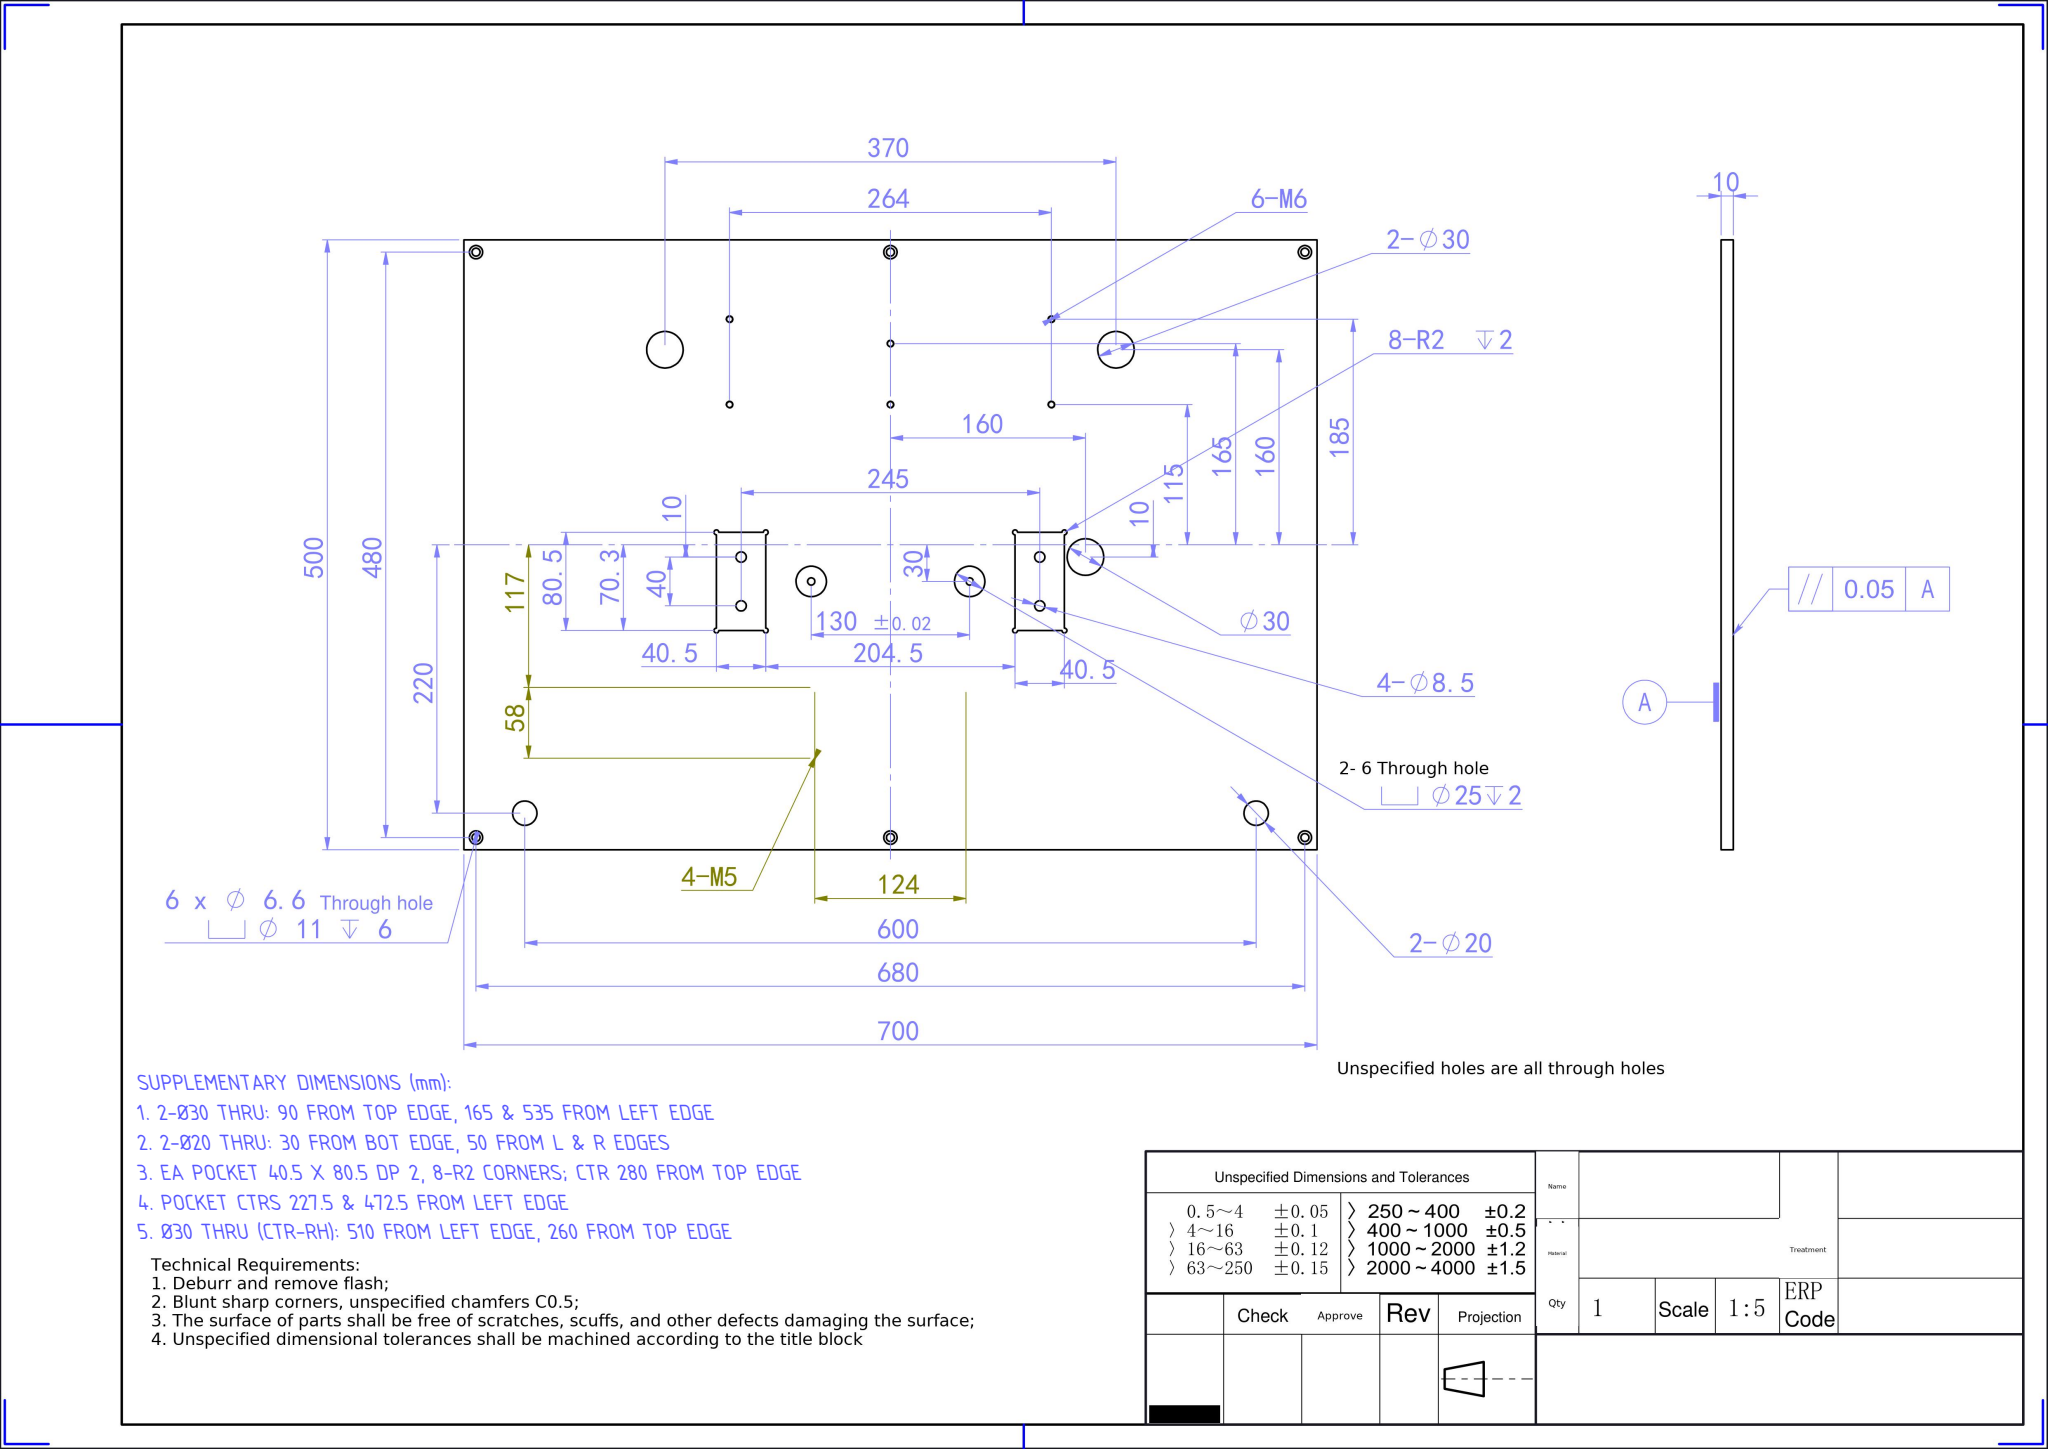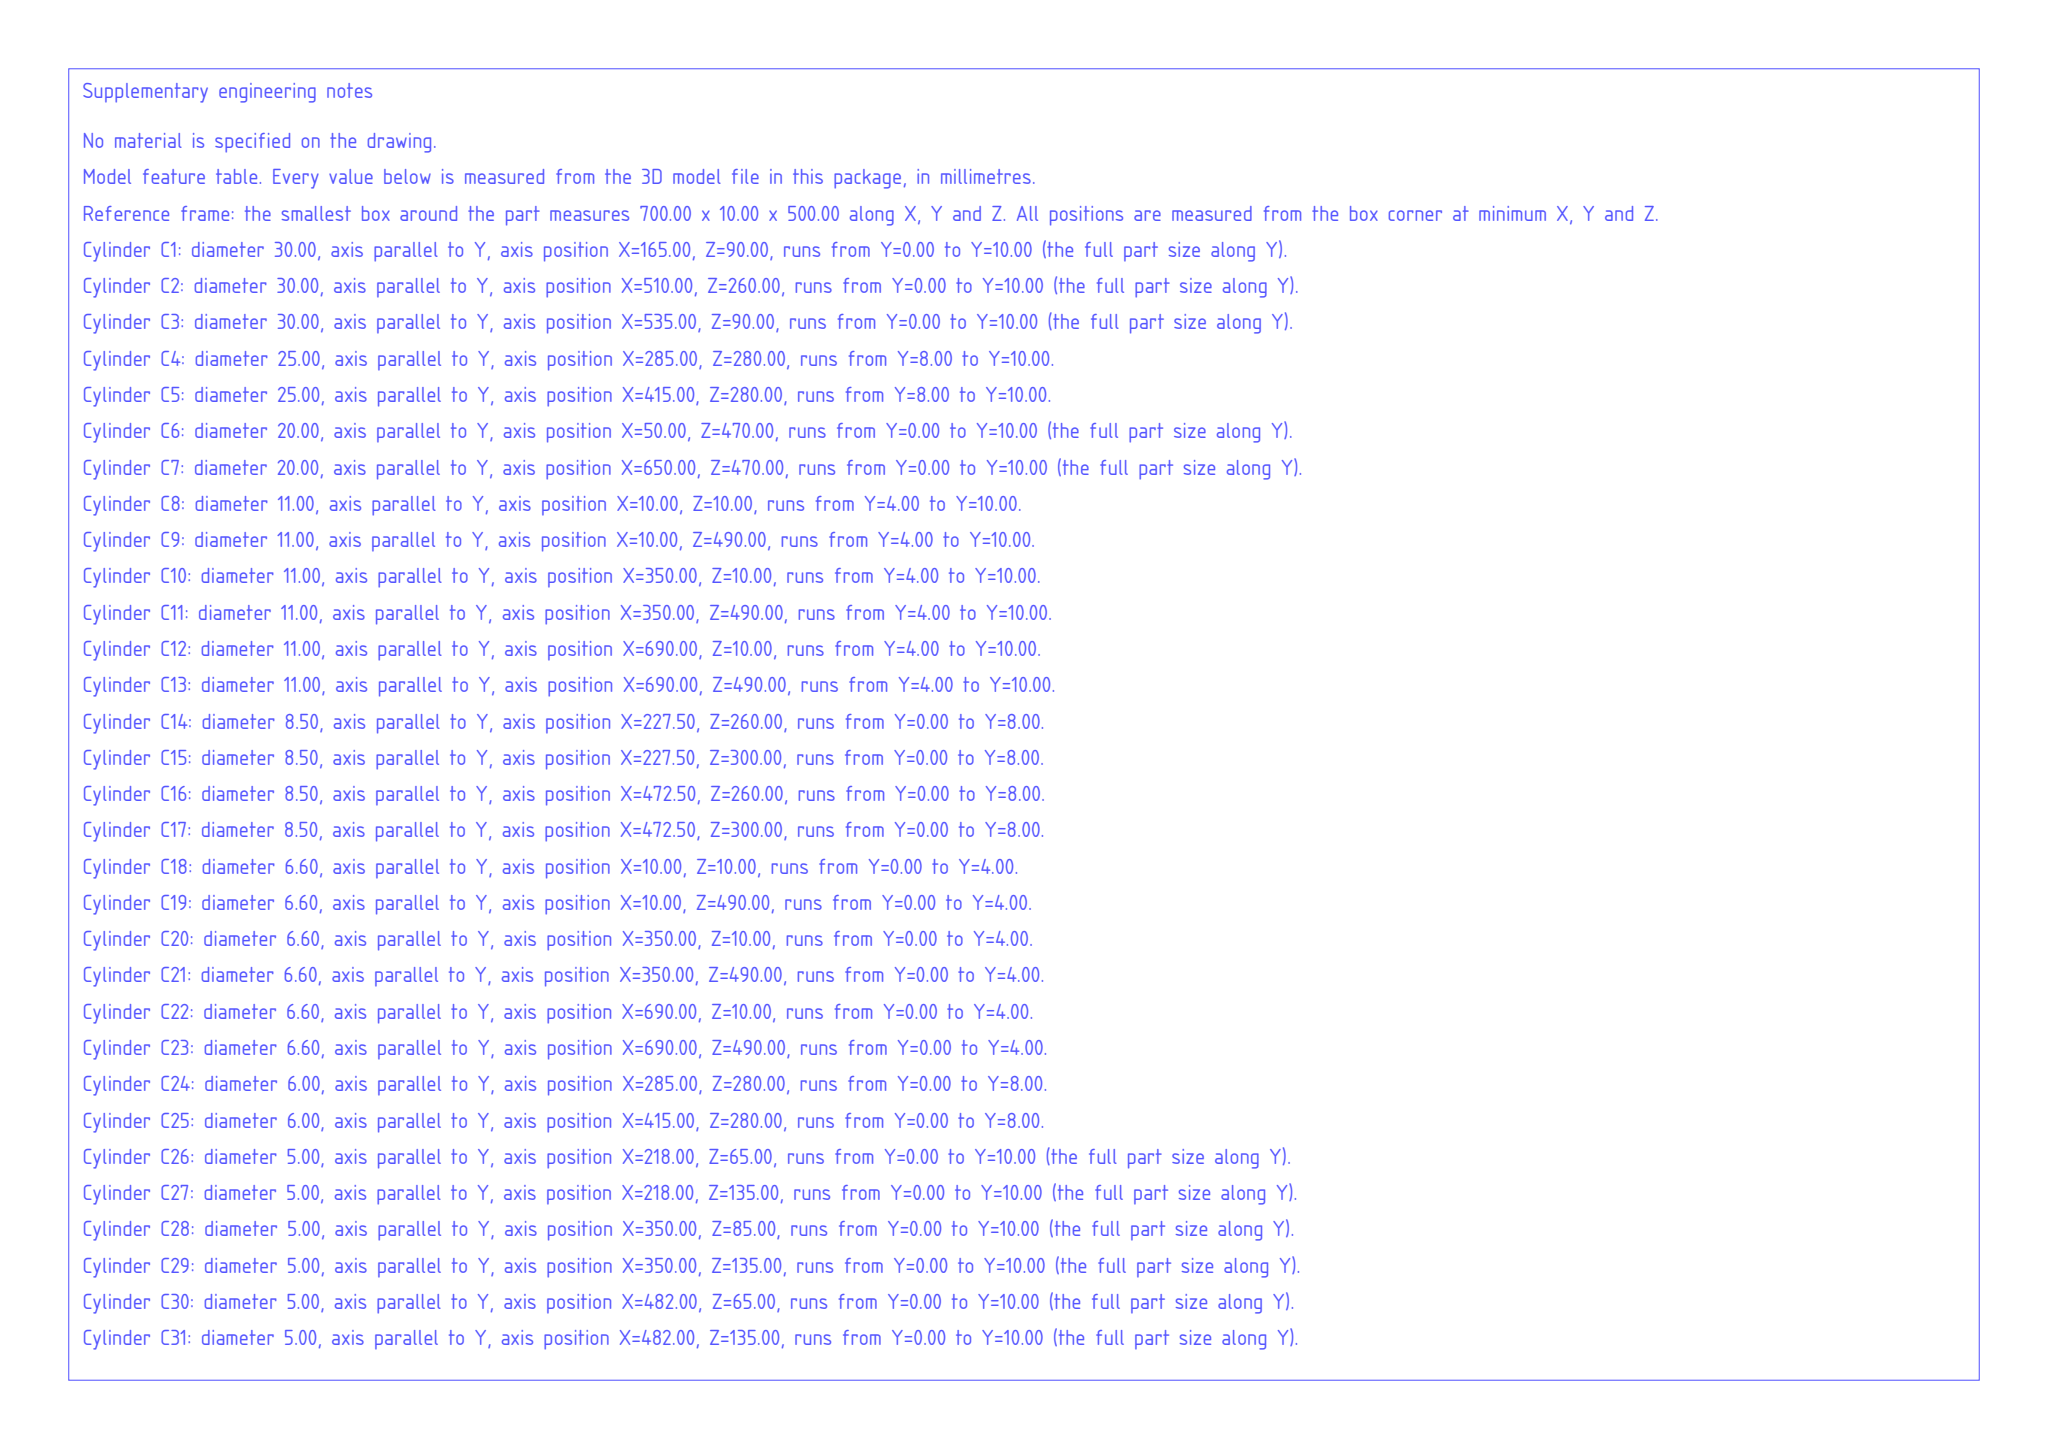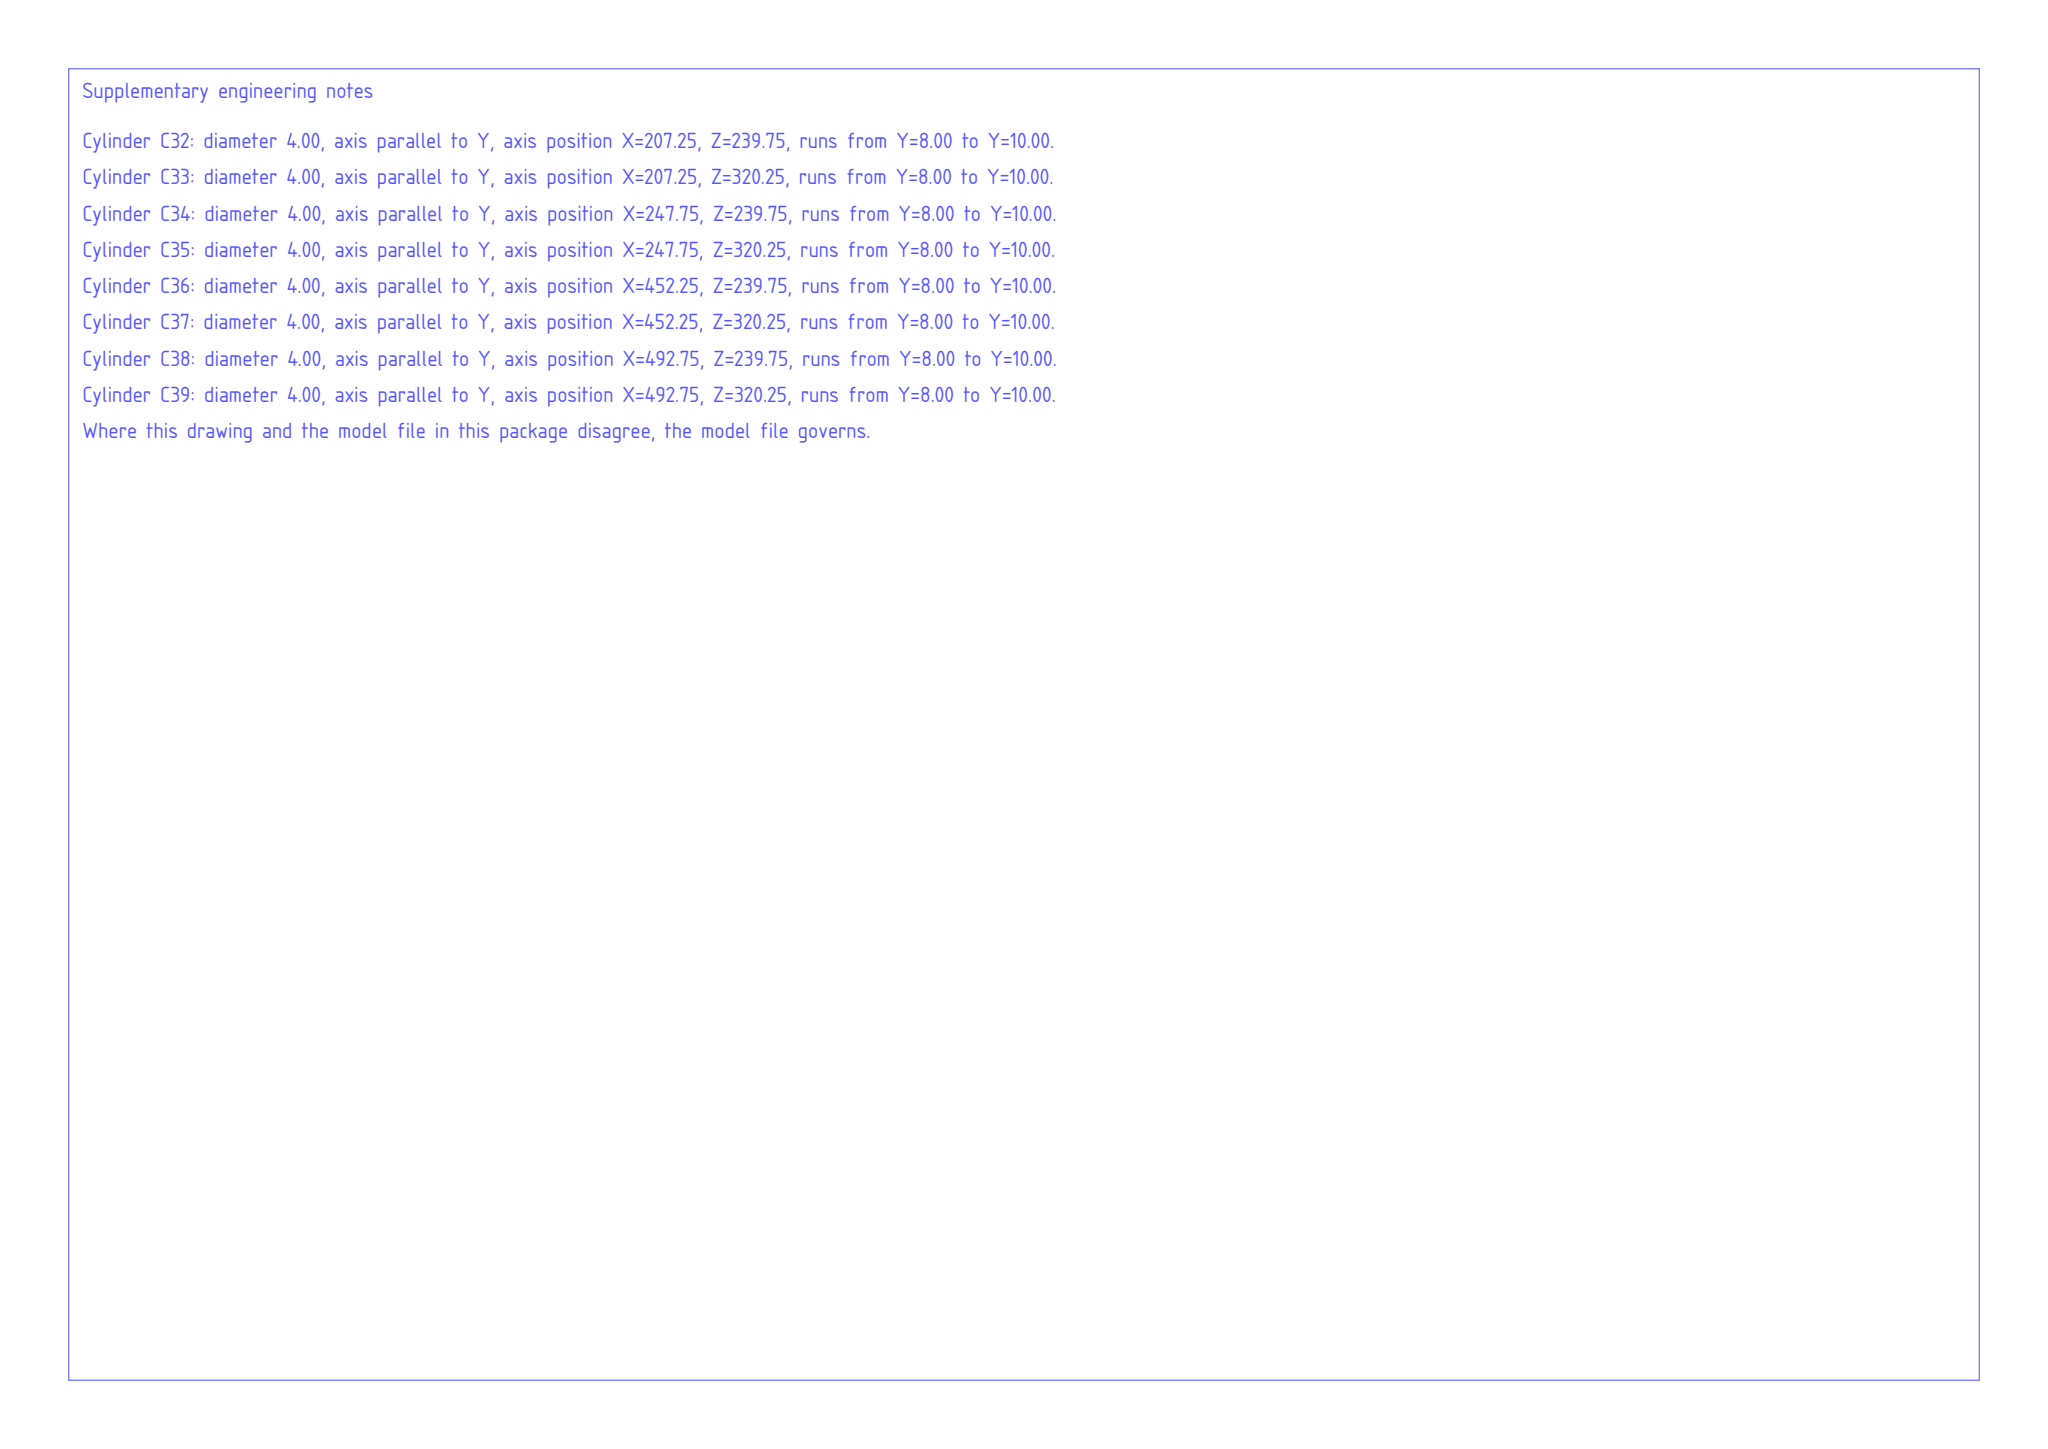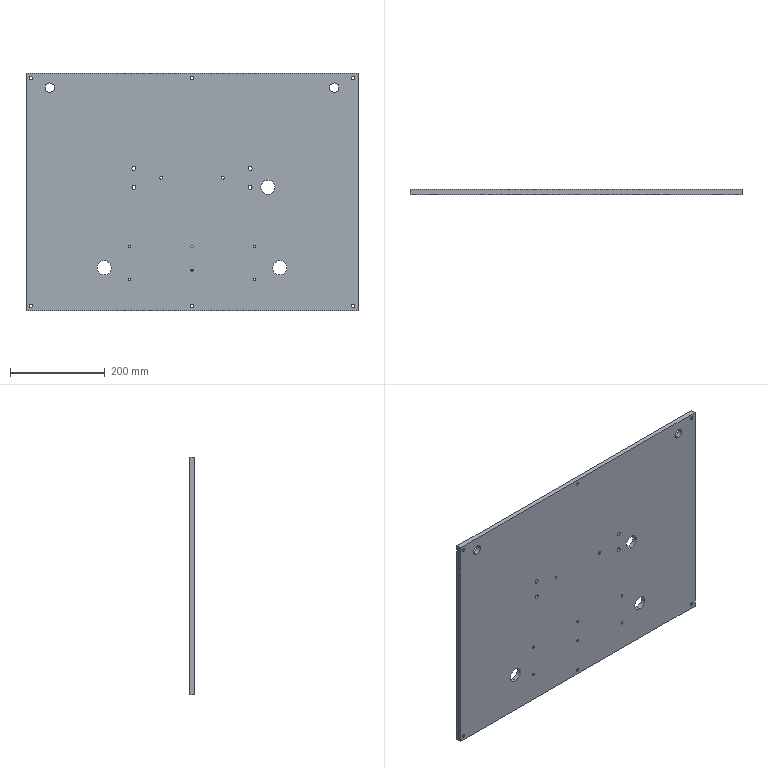Part | SolidWorks | mm | 1 solid | 98 faces | box 700 x 10 x 500 mm | volume 3449667 mm3 | cylinder 74 | plane 24 | commonest cylinder face diameters 5 x12 4 x12 11 x12 6.6 x12 8.5 x8 30 x6 6 x4 25 x4
build123d program:
from build123d import *

# Parameters (mm, degrees)
SKETCH1_W                                       = 700
SKETCH1_H                                       = 500
BOSS_EXTRUDE1_DEPTH                             = 10
M6_HEX_SOCKET_HEAD_CAP_SCREW_CBORE1_D           = 6.6
M6_HEX_SOCKET_HEAD_CAP_SCREW_CBORE1_CBORE_D     = 11
M6_HEX_SOCKET_HEAD_CAP_SCREW_CBORE1_CBORE_DEPTH = 6
F_20_0_20_DIAMETER_HOLE1_D                      = 20
SKETCH15_R                                      = 12.5
SKETCH15_W                                      = 40.5
SKETCH15_H                                      = 80.5
CUT_EXTRUDE2_DEPTH                              = 2
SKETCH16_R                                      = 2
CUT_EXTRUDE3_DEPTH                              = 2
SKETCH17_R                                      = 3
SKETCH17_R_2                                    = 4.25
CUT_EXTRUDE4_DEPTH                              = 10
SKETCH33_R                                      = 15
CUT_EXTRUDE8_DEPTH                              = 10
SKETCH37_R                                      = 15
CUT_EXTRUDE10_DEPTH                             = 20
M6_TAPPED_HOLE1_D                               = 5
M6_TAPPED_HOLE1_DEPTH                           = 17
M6_TAPPED_HOLE1_TIP                             = 1.502


with BuildPart() as part:
    # Sketch1 → Boss-Extrude1 (new body)
    with BuildSketch(Plane(origin=(0, 0, 0), x_dir=(1, 0, 0), z_dir=(0, 1, 0))):
        Rectangle(SKETCH1_W, SKETCH1_H)
    extrude(amount=BOSS_EXTRUDE1_DEPTH)

    # M6 Hex Socket Head Cap Screw CBORE1 (through all)
    with Locations(Plane(origin=(0, 10, 0), x_dir=(-1, 0, 0), z_dir=(0, 1, 0))):
        with Locations((-340, 240), (340, -240), (340, 240), (-340, -240), (0, -240), (0, 240)):
            CounterBoreHole(M6_HEX_SOCKET_HEAD_CAP_SCREW_CBORE1_D / 2, M6_HEX_SOCKET_HEAD_CAP_SCREW_CBORE1_CBORE_D / 2, M6_HEX_SOCKET_HEAD_CAP_SCREW_CBORE1_CBORE_DEPTH)

    # 20.0 _20_ Diameter Hole1 (through all)
    with Locations(Plane(origin=(0, 10, 0), x_dir=(-1, 0, 0), z_dir=(0, 1, 0))):
        with Locations((300, 220), (-300, 220)):
            Hole(F_20_0_20_DIAMETER_HOLE1_D / 2)

    # Sketch15 → Cut-Extrude2 (cut)
    with BuildSketch(Plane(origin=(0, 10, 0), x_dir=(1, 0, 0), z_dir=(0, 1, 0))):
        with Locations(Location((-65, -30, 0), (0, 0, 270))):
            Circle(SKETCH15_R)
        with Locations(Location((65, -30, 0), (0, 0, 270))):
            Circle(SKETCH15_R)
        with Locations((122.5, -30)):
            Rectangle(SKETCH15_W, SKETCH15_H)
        with Locations((-122.5, -30)):
            Rectangle(SKETCH15_W, SKETCH15_H)
    extrude(amount=-CUT_EXTRUDE2_DEPTH, mode=Mode.SUBTRACT)

    # Sketch16 → Cut-Extrude3 (cut)
    with BuildSketch(Plane(origin=(0, 10, 0), x_dir=(1, 0, 0), z_dir=(0, 1, 0))):
        with Locations((142.75, 10.25)):
            Circle(SKETCH16_R)
        with Locations((142.75, -70.25)):
            Circle(SKETCH16_R)
        with Locations((102.25, -70.25)):
            Circle(SKETCH16_R)
        with Locations((102.25, 10.25)):
            Circle(SKETCH16_R)
        with Locations((-102.25, 10.25)):
            Circle(SKETCH16_R)
        with Locations((-142.75, 10.25)):
            Circle(SKETCH16_R)
        with Locations((-102.25, -70.25)):
            Circle(SKETCH16_R)
        with Locations((-142.75, -70.25)):
            Circle(SKETCH16_R)
    extrude(amount=-CUT_EXTRUDE3_DEPTH, mode=Mode.SUBTRACT)

    # Sketch17 → Cut-Extrude4 (cut)
    with BuildSketch(Plane.XZ):
        with Locations(Location((65, 30, 0), (0, 0, 270))):
            Circle(SKETCH17_R)
        with Locations(Location((-65, 30, 0), (0, 0, 270))):
            Circle(SKETCH17_R)
        with Locations(Location((-122.5, 10, 0), (0, 0, 270))):
            Circle(SKETCH17_R_2)
        with Locations(Location((-122.5, 50, 0), (0, 0, 270))):
            Circle(SKETCH17_R_2)
        with Locations(Location((122.5, 10, 0), (0, 0, 270))):
            Circle(SKETCH17_R_2)
        with Locations(Location((122.5, 50, 0), (0, 0, 270))):
            Circle(SKETCH17_R_2)
    extrude(amount=-CUT_EXTRUDE4_DEPTH, mode=Mode.SUBTRACT)

    # Sketch33 → Cut-Extrude8 (cut)
    with BuildSketch(Plane(origin=(0, 10, 0), x_dir=(1, 0, 0), z_dir=(0, 1, 0))):
        with Locations(Location((160, -10, 0), (0, 0, 270))):
            Circle(SKETCH33_R)
    extrude(amount=-CUT_EXTRUDE8_DEPTH, mode=Mode.SUBTRACT)

    # Sketch37 → Cut-Extrude10 (cut)
    with BuildSketch(Plane(origin=(0, 10, 0), x_dir=(1, 0, 0), z_dir=(0, 1, 0))):
        with Locations(Location((185, 160, 0), (0, 0, 270))):
            Circle(SKETCH37_R)
        with Locations(Location((-185, 160, 0), (0, 0, 270))):
            Circle(SKETCH37_R)
    extrude(amount=-CUT_EXTRUDE10_DEPTH, mode=Mode.SUBTRACT)

    # M6 Tapped Hole1
    with Locations(Plane(origin=(0, 10, 0), x_dir=(1, 0, 0), z_dir=(0, 1, 0))):
        with Locations((-132, 185), (-132, 115), (0, 165), (0, 115), (132, 185), (132, 115)):
            Hole(M6_TAPPED_HOLE1_D / 2, depth=M6_TAPPED_HOLE1_DEPTH)
            with Locations((0, 0, -(M6_TAPPED_HOLE1_DEPTH + M6_TAPPED_HOLE1_TIP / 2))):  # 118° drill point
                Cone(0, M6_TAPPED_HOLE1_D / 2, M6_TAPPED_HOLE1_TIP, mode=Mode.SUBTRACT)


solid = part.part